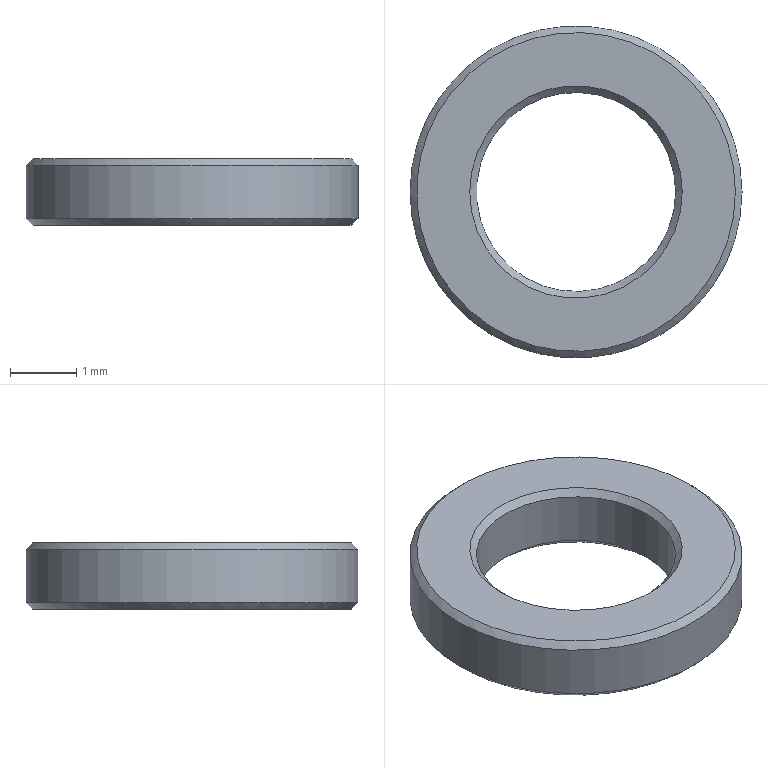Component | NX | STEPPER_WASHER | 1 solid | 15 faces | box 5 x 5 x 1 mm | volume 10 mm3 | cone 8 | cylinder 4 | plane 3 | commonest cylinder face diameters 5 x1 3 x1 4.5 x1 3.5 x1
STEP:
#1=CARTESIAN_POINT('',(0.,0.,0.));
#2=DIRECTION('',(0.,0.,1.));
#3=DIRECTION('',(1.,0.,0.));
#4=AXIS2_PLACEMENT_3D('',#1,#2,#3);
#5=CARTESIAN_POINT('',(2.4,0.,11.2));
#6=VERTEX_POINT('',#5);
#7=CARTESIAN_POINT('',(0.,0.,11.2));
#8=DIRECTION('',(0.,0.,-1.));
#9=DIRECTION('',(1.,0.,0.));
#10=AXIS2_PLACEMENT_3D('',#7,#8,#9);
#11=CIRCLE('',#10,2.4);
#12=CARTESIAN_POINT('',(0.,0.,11.2));
#13=DIRECTION('',(0.,0.,-1.));
#14=DIRECTION('',(1.,0.,0.));
#15=AXIS2_PLACEMENT_3D('',#12,#13,#14);
#16=PLANE('',#15);
#17=CARTESIAN_POINT('',(0.,0.));
#18=DIRECTION('',(1.,0.));
#19=AXIS2_PLACEMENT_2D('',#17,#18);
#20=CIRCLE('',#19,2.4);
#21=(GEOMETRIC_REPRESENTATION_CONTEXT(2)PARAMETRIC_REPRESENTATION_CONTEXT()REPRESENTATION_CONTEXT('',''));
#22=DEFINITIONAL_REPRESENTATION('',(#20),#21);
#23=PCURVE('',#16,#22);
#24=CARTESIAN_POINT('',(0.,0.,11.2));
#25=DIRECTION('',(0.,0.,1.));
#26=DIRECTION('',(-1.,0.,0.));
#27=AXIS2_PLACEMENT_3D('',#24,#25,#26);
#28=CONICAL_SURFACE('',#27,2.4,0.7854);
#29=CARTESIAN_POINT('',(9.425,0.));
#30=DIRECTION('',(-1.,0.));
#31=VECTOR('',#30,1.);
#32=LINE('',#29,#31);
#33=(GEOMETRIC_REPRESENTATION_CONTEXT(2)PARAMETRIC_REPRESENTATION_CONTEXT()REPRESENTATION_CONTEXT('',''));
#34=DEFINITIONAL_REPRESENTATION('',(#32),#33);
#35=PCURVE('',#28,#34);
#36=SURFACE_CURVE('',#11,(#23,#35),.PCURVE_S1.);
#37=EDGE_CURVE('',#6,#6,#36,.T.);
#38=ORIENTED_EDGE('',*,*,#37,.T.);
#39=EDGE_LOOP('',(#38));
#40=FACE_BOUND('',#39,.T.);
#41=CARTESIAN_POINT('',(2.35,0.,11.2));
#42=VERTEX_POINT('',#41);
#43=CARTESIAN_POINT('',(0.,0.,11.2));
#44=DIRECTION('',(0.,0.,1.));
#45=DIRECTION('',(1.,0.,0.));
#46=AXIS2_PLACEMENT_3D('',#43,#44,#45);
#47=CIRCLE('',#46,2.35);
#48=CARTESIAN_POINT('',(2.35,0.));
#49=CARTESIAN_POINT('',(2.35,-4.07));
#50=CARTESIAN_POINT('',(-1.175,-2.035));
#51=CARTESIAN_POINT('',(-4.7,-0.));
#52=CARTESIAN_POINT('',(-1.175,2.035));
#53=CARTESIAN_POINT('',(2.35,4.07));
#54=CARTESIAN_POINT('',(2.35,0.));
#55=(BOUNDED_CURVE()B_SPLINE_CURVE(2,(#48,#49,#50,#51,#52,#53,#54),.UNSPECIFIED.,.T.,.F.)B_SPLINE_CURVE_WITH_KNOTS((1,2,2,2,2,1),(-2.094,0.,2.094,4.189,6.283,8.378),.UNSPECIFIED.)CURVE()GEOMETRIC_REPRESENTATION_ITEM()RATIONAL_B_SPLINE_CURVE((1.,0.5,1.,0.5,1.,0.5,1.))REPRESENTATION_ITEM(''));
#56=(GEOMETRIC_REPRESENTATION_CONTEXT(2)PARAMETRIC_REPRESENTATION_CONTEXT()REPRESENTATION_CONTEXT('',''));
#57=DEFINITIONAL_REPRESENTATION('',(#55),#56);
#58=PCURVE('',#16,#57);
#59=CARTESIAN_POINT('',(0.,0.,11.3));
#60=DIRECTION('',(0.,0.,-1.));
#61=DIRECTION('',(1.,0.,0.));
#62=AXIS2_PLACEMENT_3D('',#59,#60,#61);
#63=CONICAL_SURFACE('',#62,2.25,0.7854);
#64=CARTESIAN_POINT('',(6.283,0.1));
#65=DIRECTION('',(-1.,0.));
#66=VECTOR('',#65,1.);
#67=LINE('',#64,#66);
#68=(GEOMETRIC_REPRESENTATION_CONTEXT(2)PARAMETRIC_REPRESENTATION_CONTEXT()REPRESENTATION_CONTEXT('',''));
#69=DEFINITIONAL_REPRESENTATION('',(#67),#68);
#70=PCURVE('',#63,#69);
#71=SURFACE_CURVE('',#47,(#58,#70),.PCURVE_S1.);
#72=EDGE_CURVE('',#42,#42,#71,.T.);
#73=ORIENTED_EDGE('',*,*,#72,.T.);
#74=EDGE_LOOP('',(#73));
#75=FACE_BOUND('',#74,.T.);
#76=ADVANCED_FACE('',(#40,#75),#16,.T.);
#77=CARTESIAN_POINT('',(2.5,0.,12.1));
#78=VERTEX_POINT('',#77);
#79=CARTESIAN_POINT('',(0.,0.,12.1));
#80=DIRECTION('',(0.,0.,-1.));
#81=DIRECTION('',(1.,0.,0.));
#82=AXIS2_PLACEMENT_3D('',#79,#80,#81);
#83=CIRCLE('',#82,2.5);
#84=CARTESIAN_POINT('',(0.,0.,11.2));
#85=DIRECTION('',(0.,0.,1.));
#86=DIRECTION('',(-1.,0.,0.));
#87=AXIS2_PLACEMENT_3D('',#84,#85,#86);
#88=CYLINDRICAL_SURFACE('',#87,2.5);
#89=CARTESIAN_POINT('',(9.425,0.9));
#90=DIRECTION('',(-1.,0.));
#91=VECTOR('',#90,1.);
#92=LINE('',#89,#91);
#93=(GEOMETRIC_REPRESENTATION_CONTEXT(2)PARAMETRIC_REPRESENTATION_CONTEXT()REPRESENTATION_CONTEXT('',''));
#94=DEFINITIONAL_REPRESENTATION('',(#92),#93);
#95=PCURVE('',#88,#94);
#96=CARTESIAN_POINT('',(0.,0.,12.1));
#97=DIRECTION('',(0.,0.,-1.));
#98=DIRECTION('',(1.,0.,0.));
#99=AXIS2_PLACEMENT_3D('',#96,#97,#98);
#100=CONICAL_SURFACE('',#99,2.5,0.7854);
#101=CARTESIAN_POINT('',(0.,0.));
#102=DIRECTION('',(1.,0.));
#103=VECTOR('',#102,1.);
#104=LINE('',#101,#103);
#105=(GEOMETRIC_REPRESENTATION_CONTEXT(2)PARAMETRIC_REPRESENTATION_CONTEXT()REPRESENTATION_CONTEXT('',''));
#106=DEFINITIONAL_REPRESENTATION('',(#104),#105);
#107=PCURVE('',#100,#106);
#108=SURFACE_CURVE('',#83,(#95,#107),.PCURVE_S1.);
#109=EDGE_CURVE('',#78,#78,#108,.T.);
#110=ORIENTED_EDGE('',*,*,#109,.T.);
#111=CARTESIAN_POINT('',(2.5,0.,11.3));
#112=VERTEX_POINT('',#111);
#113=CARTESIAN_POINT('',(2.5,-0.,11.3));
#114=CARTESIAN_POINT('',(2.5,-0.,12.1));
#115=B_SPLINE_CURVE_WITH_KNOTS('',1,(#113,#114),.UNSPECIFIED.,.F.,.F.,(2,2),(0.1,0.9),.PIECEWISE_BEZIER_KNOTS.);
#116=CARTESIAN_POINT('',(3.142,0.));
#117=DIRECTION('',(0.,1.));
#118=VECTOR('',#117,1.);
#119=LINE('',#116,#118);
#120=(GEOMETRIC_REPRESENTATION_CONTEXT(2)PARAMETRIC_REPRESENTATION_CONTEXT()REPRESENTATION_CONTEXT('',''));
#121=DEFINITIONAL_REPRESENTATION('',(#119),#120);
#122=PCURVE('',#88,#121);
#123=CARTESIAN_POINT('',(9.425,0.));
#124=DIRECTION('',(0.,1.));
#125=VECTOR('',#124,1.);
#126=LINE('',#123,#125);
#127=(GEOMETRIC_REPRESENTATION_CONTEXT(2)PARAMETRIC_REPRESENTATION_CONTEXT()REPRESENTATION_CONTEXT('',''));
#128=DEFINITIONAL_REPRESENTATION('',(#126),#127);
#129=PCURVE('',#88,#128);
#130=SEAM_CURVE('',#115,(#122,#129),.PCURVE_S1.);
#131=EDGE_CURVE('',#112,#78,#130,.T.);
#132=ORIENTED_EDGE('',*,*,#131,.F.);
#133=CARTESIAN_POINT('',(0.,0.,11.3));
#134=DIRECTION('',(0.,0.,1.));
#135=DIRECTION('',(1.,0.,0.));
#136=AXIS2_PLACEMENT_3D('',#133,#134,#135);
#137=CIRCLE('',#136,2.5);
#138=CARTESIAN_POINT('',(3.142,0.1));
#139=DIRECTION('',(1.,0.));
#140=VECTOR('',#139,1.);
#141=LINE('',#138,#140);
#142=(GEOMETRIC_REPRESENTATION_CONTEXT(2)PARAMETRIC_REPRESENTATION_CONTEXT()REPRESENTATION_CONTEXT('',''));
#143=DEFINITIONAL_REPRESENTATION('',(#141),#142);
#144=PCURVE('',#88,#143);
#145=CARTESIAN_POINT('',(3.142,0.1));
#146=DIRECTION('',(1.,0.));
#147=VECTOR('',#146,1.);
#148=LINE('',#145,#147);
#149=(GEOMETRIC_REPRESENTATION_CONTEXT(2)PARAMETRIC_REPRESENTATION_CONTEXT()REPRESENTATION_CONTEXT('',''));
#150=DEFINITIONAL_REPRESENTATION('',(#148),#149);
#151=PCURVE('',#28,#150);
#152=SURFACE_CURVE('',#137,(#144,#151),.PCURVE_S1.);
#153=EDGE_CURVE('',#112,#112,#152,.T.);
#154=ORIENTED_EDGE('',*,*,#153,.T.);
#155=ORIENTED_EDGE('',*,*,#131,.T.);
#156=EDGE_LOOP('',(#110,#132,#154,#155));
#157=FACE_BOUND('',#156,.T.);
#158=ADVANCED_FACE('',(#157),#88,.T.);
#159=CARTESIAN_POINT('',(1.5,0.,12.1));
#160=VERTEX_POINT('',#159);
#161=CARTESIAN_POINT('',(0.,0.,12.1));
#162=DIRECTION('',(0.,0.,1.));
#163=DIRECTION('',(1.,0.,0.));
#164=AXIS2_PLACEMENT_3D('',#161,#162,#163);
#165=CIRCLE('',#164,1.5);
#166=CARTESIAN_POINT('',(0.,0.,11.2));
#167=DIRECTION('',(0.,0.,1.));
#168=DIRECTION('',(-1.,0.,0.));
#169=AXIS2_PLACEMENT_3D('',#166,#167,#168);
#170=CYLINDRICAL_SURFACE('',#169,1.5);
#171=CARTESIAN_POINT('',(3.142,0.9));
#172=DIRECTION('',(1.,0.));
#173=VECTOR('',#172,1.);
#174=LINE('',#171,#173);
#175=(GEOMETRIC_REPRESENTATION_CONTEXT(2)PARAMETRIC_REPRESENTATION_CONTEXT()REPRESENTATION_CONTEXT('',''));
#176=DEFINITIONAL_REPRESENTATION('',(#174),#175);
#177=PCURVE('',#170,#176);
#178=CARTESIAN_POINT('',(0.,0.,12.2));
#179=DIRECTION('',(0.,0.,1.));
#180=DIRECTION('',(-1.,0.,0.));
#181=AXIS2_PLACEMENT_3D('',#178,#179,#180);
#182=CONICAL_SURFACE('',#181,1.6,0.7854);
#183=CARTESIAN_POINT('',(3.142,-0.1));
#184=DIRECTION('',(1.,0.));
#185=VECTOR('',#184,1.);
#186=LINE('',#183,#185);
#187=(GEOMETRIC_REPRESENTATION_CONTEXT(2)PARAMETRIC_REPRESENTATION_CONTEXT()REPRESENTATION_CONTEXT('',''));
#188=DEFINITIONAL_REPRESENTATION('',(#186),#187);
#189=PCURVE('',#182,#188);
#190=SURFACE_CURVE('',#165,(#177,#189),.PCURVE_S1.);
#191=EDGE_CURVE('',#160,#160,#190,.T.);
#192=ORIENTED_EDGE('',*,*,#191,.F.);
#193=CARTESIAN_POINT('',(1.5,0.,11.3));
#194=VERTEX_POINT('',#193);
#195=CARTESIAN_POINT('',(1.5,-0.,11.3));
#196=CARTESIAN_POINT('',(1.5,-0.,12.1));
#197=B_SPLINE_CURVE_WITH_KNOTS('',1,(#195,#196),.UNSPECIFIED.,.F.,.F.,(2,2),(0.1,0.9),.PIECEWISE_BEZIER_KNOTS.);
#198=CARTESIAN_POINT('',(3.142,0.));
#199=DIRECTION('',(0.,1.));
#200=VECTOR('',#199,1.);
#201=LINE('',#198,#200);
#202=(GEOMETRIC_REPRESENTATION_CONTEXT(2)PARAMETRIC_REPRESENTATION_CONTEXT()REPRESENTATION_CONTEXT('',''));
#203=DEFINITIONAL_REPRESENTATION('',(#201),#202);
#204=PCURVE('',#170,#203);
#205=CARTESIAN_POINT('',(9.425,0.));
#206=DIRECTION('',(0.,1.));
#207=VECTOR('',#206,1.);
#208=LINE('',#205,#207);
#209=(GEOMETRIC_REPRESENTATION_CONTEXT(2)PARAMETRIC_REPRESENTATION_CONTEXT()REPRESENTATION_CONTEXT('',''));
#210=DEFINITIONAL_REPRESENTATION('',(#208),#209);
#211=PCURVE('',#170,#210);
#212=SEAM_CURVE('',#197,(#204,#211),.PCURVE_S1.);
#213=EDGE_CURVE('',#194,#160,#212,.T.);
#214=ORIENTED_EDGE('',*,*,#213,.F.);
#215=CARTESIAN_POINT('',(0.,0.,11.3));
#216=DIRECTION('',(0.,0.,-1.));
#217=DIRECTION('',(1.,0.,0.));
#218=AXIS2_PLACEMENT_3D('',#215,#216,#217);
#219=CIRCLE('',#218,1.5);
#220=CARTESIAN_POINT('',(9.425,0.1));
#221=DIRECTION('',(-1.,0.));
#222=VECTOR('',#221,1.);
#223=LINE('',#220,#222);
#224=(GEOMETRIC_REPRESENTATION_CONTEXT(2)PARAMETRIC_REPRESENTATION_CONTEXT()REPRESENTATION_CONTEXT('',''));
#225=DEFINITIONAL_REPRESENTATION('',(#223),#224);
#226=PCURVE('',#170,#225);
#227=CARTESIAN_POINT('',(0.,0.,11.3));
#228=DIRECTION('',(0.,0.,-1.));
#229=DIRECTION('',(1.,0.,0.));
#230=AXIS2_PLACEMENT_3D('',#227,#228,#229);
#231=CONICAL_SURFACE('',#230,1.5,0.7854);
#232=CARTESIAN_POINT('',(0.,0.));
#233=DIRECTION('',(1.,0.));
#234=VECTOR('',#233,1.);
#235=LINE('',#232,#234);
#236=(GEOMETRIC_REPRESENTATION_CONTEXT(2)PARAMETRIC_REPRESENTATION_CONTEXT()REPRESENTATION_CONTEXT('',''));
#237=DEFINITIONAL_REPRESENTATION('',(#235),#236);
#238=PCURVE('',#231,#237);
#239=SURFACE_CURVE('',#219,(#226,#238),.PCURVE_S1.);
#240=EDGE_CURVE('',#194,#194,#239,.T.);
#241=ORIENTED_EDGE('',*,*,#240,.F.);
#242=ORIENTED_EDGE('',*,*,#213,.T.);
#243=EDGE_LOOP('',(#192,#214,#241,#242));
#244=FACE_BOUND('',#243,.F.);
#245=ADVANCED_FACE('',(#244),#170,.F.);
#246=CARTESIAN_POINT('',(1.6,0.,11.2));
#247=VERTEX_POINT('',#246);
#248=CARTESIAN_POINT('',(0.,0.,11.2));
#249=DIRECTION('',(0.,0.,1.));
#250=DIRECTION('',(1.,0.,0.));
#251=AXIS2_PLACEMENT_3D('',#248,#249,#250);
#252=CIRCLE('',#251,1.6);
#253=CARTESIAN_POINT('',(0.,0.,11.2));
#254=DIRECTION('',(0.,0.,-1.));
#255=DIRECTION('',(1.,0.,0.));
#256=AXIS2_PLACEMENT_3D('',#253,#254,#255);
#257=PLANE('',#256);
#258=CARTESIAN_POINT('',(1.6,0.));
#259=CARTESIAN_POINT('',(1.6,-2.771));
#260=CARTESIAN_POINT('',(-0.8,-1.386));
#261=CARTESIAN_POINT('',(-3.2,-0.));
#262=CARTESIAN_POINT('',(-0.8,1.386));
#263=CARTESIAN_POINT('',(1.6,2.771));
#264=CARTESIAN_POINT('',(1.6,0.));
#265=(BOUNDED_CURVE()B_SPLINE_CURVE(2,(#258,#259,#260,#261,#262,#263,#264),.UNSPECIFIED.,.T.,.F.)B_SPLINE_CURVE_WITH_KNOTS((1,2,2,2,2,1),(-2.094,0.,2.094,4.189,6.283,8.378),.UNSPECIFIED.)CURVE()GEOMETRIC_REPRESENTATION_ITEM()RATIONAL_B_SPLINE_CURVE((1.,0.5,1.,0.5,1.,0.5,1.))REPRESENTATION_ITEM(''));
#266=(GEOMETRIC_REPRESENTATION_CONTEXT(2)PARAMETRIC_REPRESENTATION_CONTEXT()REPRESENTATION_CONTEXT('',''));
#267=DEFINITIONAL_REPRESENTATION('',(#265),#266);
#268=PCURVE('',#257,#267);
#269=CARTESIAN_POINT('',(6.283,0.1));
#270=DIRECTION('',(-1.,0.));
#271=VECTOR('',#270,1.);
#272=LINE('',#269,#271);
#273=(GEOMETRIC_REPRESENTATION_CONTEXT(2)PARAMETRIC_REPRESENTATION_CONTEXT()REPRESENTATION_CONTEXT('',''));
#274=DEFINITIONAL_REPRESENTATION('',(#272),#273);
#275=PCURVE('',#231,#274);
#276=SURFACE_CURVE('',#252,(#268,#275),.PCURVE_S1.);
#277=EDGE_CURVE('',#247,#247,#276,.T.);
#278=ORIENTED_EDGE('',*,*,#277,.T.);
#279=EDGE_LOOP('',(#278));
#280=FACE_BOUND('',#279,.T.);
#281=CARTESIAN_POINT('',(1.65,0.,11.2));
#282=VERTEX_POINT('',#281);
#283=CARTESIAN_POINT('',(0.,0.,11.2));
#284=DIRECTION('',(0.,0.,-1.));
#285=DIRECTION('',(1.,0.,0.));
#286=AXIS2_PLACEMENT_3D('',#283,#284,#285);
#287=CIRCLE('',#286,1.65);
#288=CARTESIAN_POINT('',(0.,0.));
#289=DIRECTION('',(1.,0.));
#290=AXIS2_PLACEMENT_2D('',#288,#289);
#291=CIRCLE('',#290,1.65);
#292=(GEOMETRIC_REPRESENTATION_CONTEXT(2)PARAMETRIC_REPRESENTATION_CONTEXT()REPRESENTATION_CONTEXT('',''));
#293=DEFINITIONAL_REPRESENTATION('',(#291),#292);
#294=PCURVE('',#257,#293);
#295=CARTESIAN_POINT('',(0.,0.,11.3));
#296=DIRECTION('',(0.,0.,1.));
#297=DIRECTION('',(-1.,0.,0.));
#298=AXIS2_PLACEMENT_3D('',#295,#296,#297);
#299=CONICAL_SURFACE('',#298,1.75,0.7854);
#300=CARTESIAN_POINT('',(9.425,-0.1));
#301=DIRECTION('',(-1.,0.));
#302=VECTOR('',#301,1.);
#303=LINE('',#300,#302);
#304=(GEOMETRIC_REPRESENTATION_CONTEXT(2)PARAMETRIC_REPRESENTATION_CONTEXT()REPRESENTATION_CONTEXT('',''));
#305=DEFINITIONAL_REPRESENTATION('',(#303),#304);
#306=PCURVE('',#299,#305);
#307=SURFACE_CURVE('',#287,(#294,#306),.PCURVE_S1.);
#308=EDGE_CURVE('',#282,#282,#307,.T.);
#309=ORIENTED_EDGE('',*,*,#308,.T.);
#310=EDGE_LOOP('',(#309));
#311=FACE_BOUND('',#310,.T.);
#312=ADVANCED_FACE('',(#280,#311),#257,.T.);
#313=CARTESIAN_POINT('',(1.6,0.,12.2));
#314=VERTEX_POINT('',#313);
#315=CARTESIAN_POINT('',(0.,0.,12.2));
#316=DIRECTION('',(0.,0.,-1.));
#317=DIRECTION('',(1.,0.,0.));
#318=AXIS2_PLACEMENT_3D('',#315,#316,#317);
#319=CIRCLE('',#318,1.6);
#320=CARTESIAN_POINT('',(0.,0.,12.2));
#321=DIRECTION('',(0.,0.,-1.));
#322=DIRECTION('',(1.,0.,0.));
#323=AXIS2_PLACEMENT_3D('',#320,#321,#322);
#324=PLANE('',#323);
#325=CARTESIAN_POINT('',(0.,0.));
#326=DIRECTION('',(1.,0.));
#327=AXIS2_PLACEMENT_2D('',#325,#326);
#328=CIRCLE('',#327,1.6);
#329=(GEOMETRIC_REPRESENTATION_CONTEXT(2)PARAMETRIC_REPRESENTATION_CONTEXT()REPRESENTATION_CONTEXT('',''));
#330=DEFINITIONAL_REPRESENTATION('',(#328),#329);
#331=PCURVE('',#324,#330);
#332=CARTESIAN_POINT('',(9.425,0.));
#333=DIRECTION('',(-1.,0.));
#334=VECTOR('',#333,1.);
#335=LINE('',#332,#334);
#336=(GEOMETRIC_REPRESENTATION_CONTEXT(2)PARAMETRIC_REPRESENTATION_CONTEXT()REPRESENTATION_CONTEXT('',''));
#337=DEFINITIONAL_REPRESENTATION('',(#335),#336);
#338=PCURVE('',#182,#337);
#339=SURFACE_CURVE('',#319,(#331,#338),.PCURVE_S1.);
#340=EDGE_CURVE('',#314,#314,#339,.T.);
#341=ORIENTED_EDGE('',*,*,#340,.T.);
#342=EDGE_LOOP('',(#341));
#343=FACE_BOUND('',#342,.T.);
#344=CARTESIAN_POINT('',(2.4,0.,12.2));
#345=VERTEX_POINT('',#344);
#346=CARTESIAN_POINT('',(0.,0.,12.2));
#347=DIRECTION('',(0.,0.,1.));
#348=DIRECTION('',(1.,0.,0.));
#349=AXIS2_PLACEMENT_3D('',#346,#347,#348);
#350=CIRCLE('',#349,2.4);
#351=CARTESIAN_POINT('',(2.4,0.));
#352=CARTESIAN_POINT('',(2.4,-4.157));
#353=CARTESIAN_POINT('',(-1.2,-2.078));
#354=CARTESIAN_POINT('',(-4.8,-0.));
#355=CARTESIAN_POINT('',(-1.2,2.078));
#356=CARTESIAN_POINT('',(2.4,4.157));
#357=CARTESIAN_POINT('',(2.4,0.));
#358=(BOUNDED_CURVE()B_SPLINE_CURVE(2,(#351,#352,#353,#354,#355,#356,#357),.UNSPECIFIED.,.T.,.F.)B_SPLINE_CURVE_WITH_KNOTS((1,2,2,2,2,1),(-2.094,0.,2.094,4.189,6.283,8.378),.UNSPECIFIED.)CURVE()GEOMETRIC_REPRESENTATION_ITEM()RATIONAL_B_SPLINE_CURVE((1.,0.5,1.,0.5,1.,0.5,1.))REPRESENTATION_ITEM(''));
#359=(GEOMETRIC_REPRESENTATION_CONTEXT(2)PARAMETRIC_REPRESENTATION_CONTEXT()REPRESENTATION_CONTEXT('',''));
#360=DEFINITIONAL_REPRESENTATION('',(#358),#359);
#361=PCURVE('',#324,#360);
#362=CARTESIAN_POINT('',(6.283,-0.1));
#363=DIRECTION('',(-1.,0.));
#364=VECTOR('',#363,1.);
#365=LINE('',#362,#364);
#366=(GEOMETRIC_REPRESENTATION_CONTEXT(2)PARAMETRIC_REPRESENTATION_CONTEXT()REPRESENTATION_CONTEXT('',''));
#367=DEFINITIONAL_REPRESENTATION('',(#365),#366);
#368=PCURVE('',#100,#367);
#369=SURFACE_CURVE('',#350,(#361,#368),.PCURVE_S1.);
#370=EDGE_CURVE('',#345,#345,#369,.T.);
#371=ORIENTED_EDGE('',*,*,#370,.T.);
#372=EDGE_LOOP('',(#371));
#373=FACE_BOUND('',#372,.T.);
#374=ADVANCED_FACE('',(#343,#373),#324,.F.);
#375=CARTESIAN_POINT('',(2.25,0.,11.3));
#376=VERTEX_POINT('',#375);
#377=CARTESIAN_POINT('',(0.,0.,11.3));
#378=DIRECTION('',(0.,0.,-1.));
#379=DIRECTION('',(1.,0.,0.));
#380=AXIS2_PLACEMENT_3D('',#377,#378,#379);
#381=CIRCLE('',#380,2.25);
#382=CARTESIAN_POINT('',(0.,0.,11.7));
#383=DIRECTION('',(0.,0.,-1.));
#384=DIRECTION('',(1.,0.,0.));
#385=AXIS2_PLACEMENT_3D('',#382,#383,#384);
#386=CYLINDRICAL_SURFACE('',#385,2.25);
#387=CARTESIAN_POINT('',(0.,0.4));
#388=DIRECTION('',(1.,0.));
#389=VECTOR('',#388,1.);
#390=LINE('',#387,#389);
#391=(GEOMETRIC_REPRESENTATION_CONTEXT(2)PARAMETRIC_REPRESENTATION_CONTEXT()REPRESENTATION_CONTEXT('',''));
#392=DEFINITIONAL_REPRESENTATION('',(#390),#391);
#393=PCURVE('',#386,#392);
#394=CARTESIAN_POINT('',(0.,0.));
#395=DIRECTION('',(1.,0.));
#396=VECTOR('',#395,1.);
#397=LINE('',#394,#396);
#398=(GEOMETRIC_REPRESENTATION_CONTEXT(2)PARAMETRIC_REPRESENTATION_CONTEXT()REPRESENTATION_CONTEXT('',''));
#399=DEFINITIONAL_REPRESENTATION('',(#397),#398);
#400=PCURVE('',#63,#399);
#401=SURFACE_CURVE('',#381,(#393,#400),.PCURVE_S1.);
#402=EDGE_CURVE('',#376,#376,#401,.T.);
#403=ORIENTED_EDGE('',*,*,#402,.F.);
#404=CARTESIAN_POINT('',(2.25,0.,11.45));
#405=VERTEX_POINT('',#404);
#406=CARTESIAN_POINT('',(2.25,0.,11.45));
#407=CARTESIAN_POINT('',(2.25,0.,11.3));
#408=B_SPLINE_CURVE_WITH_KNOTS('',1,(#406,#407),.UNSPECIFIED.,.F.,.F.,(2,2),(0.25,0.4),.PIECEWISE_BEZIER_KNOTS.);
#409=CARTESIAN_POINT('',(0.,0.));
#410=DIRECTION('',(0.,1.));
#411=VECTOR('',#410,1.);
#412=LINE('',#409,#411);
#413=(GEOMETRIC_REPRESENTATION_CONTEXT(2)PARAMETRIC_REPRESENTATION_CONTEXT()REPRESENTATION_CONTEXT('',''));
#414=DEFINITIONAL_REPRESENTATION('',(#412),#413);
#415=PCURVE('',#386,#414);
#416=CARTESIAN_POINT('',(6.283,0.));
#417=DIRECTION('',(0.,1.));
#418=VECTOR('',#417,1.);
#419=LINE('',#416,#418);
#420=(GEOMETRIC_REPRESENTATION_CONTEXT(2)PARAMETRIC_REPRESENTATION_CONTEXT()REPRESENTATION_CONTEXT('',''));
#421=DEFINITIONAL_REPRESENTATION('',(#419),#420);
#422=PCURVE('',#386,#421);
#423=SEAM_CURVE('',#408,(#415,#422),.PCURVE_S1.);
#424=EDGE_CURVE('',#405,#376,#423,.T.);
#425=ORIENTED_EDGE('',*,*,#424,.F.);
#426=CARTESIAN_POINT('',(0.,0.,11.45));
#427=DIRECTION('',(0.,0.,1.));
#428=DIRECTION('',(1.,0.,0.));
#429=AXIS2_PLACEMENT_3D('',#426,#427,#428);
#430=CIRCLE('',#429,2.25);
#431=CARTESIAN_POINT('',(6.283,0.25));
#432=DIRECTION('',(-1.,0.));
#433=VECTOR('',#432,1.);
#434=LINE('',#431,#433);
#435=(GEOMETRIC_REPRESENTATION_CONTEXT(2)PARAMETRIC_REPRESENTATION_CONTEXT()REPRESENTATION_CONTEXT('',''));
#436=DEFINITIONAL_REPRESENTATION('',(#434),#435);
#437=PCURVE('',#386,#436);
#438=CARTESIAN_POINT('',(0.,0.,11.45));
#439=DIRECTION('',(0.,0.,-1.));
#440=DIRECTION('',(1.,0.,0.));
#441=AXIS2_PLACEMENT_3D('',#438,#439,#440);
#442=CONICAL_SURFACE('',#441,2.25,0.7854);
#443=CARTESIAN_POINT('',(6.283,0.));
#444=DIRECTION('',(-1.,0.));
#445=VECTOR('',#444,1.);
#446=LINE('',#443,#445);
#447=(GEOMETRIC_REPRESENTATION_CONTEXT(2)PARAMETRIC_REPRESENTATION_CONTEXT()REPRESENTATION_CONTEXT('',''));
#448=DEFINITIONAL_REPRESENTATION('',(#446),#447);
#449=PCURVE('',#442,#448);
#450=SURFACE_CURVE('',#430,(#437,#449),.PCURVE_S1.);
#451=EDGE_CURVE('',#405,#405,#450,.T.);
#452=ORIENTED_EDGE('',*,*,#451,.F.);
#453=ORIENTED_EDGE('',*,*,#424,.T.);
#454=EDGE_LOOP('',(#403,#425,#452,#453));
#455=FACE_BOUND('',#454,.F.);
#456=ADVANCED_FACE('',(#455),#386,.F.);
#457=CARTESIAN_POINT('',(1.75,0.,11.3));
#458=VERTEX_POINT('',#457);
#459=CARTESIAN_POINT('',(0.,0.,11.3));
#460=DIRECTION('',(0.,0.,1.));
#461=DIRECTION('',(1.,0.,0.));
#462=AXIS2_PLACEMENT_3D('',#459,#460,#461);
#463=CIRCLE('',#462,1.75);
#464=CARTESIAN_POINT('',(0.,0.,11.7));
#465=DIRECTION('',(0.,0.,-1.));
#466=DIRECTION('',(1.,0.,0.));
#467=AXIS2_PLACEMENT_3D('',#464,#465,#466);
#468=CYLINDRICAL_SURFACE('',#467,1.75);
#469=CARTESIAN_POINT('',(6.283,0.4));
#470=DIRECTION('',(-1.,0.));
#471=VECTOR('',#470,1.);
#472=LINE('',#469,#471);
#473=(GEOMETRIC_REPRESENTATION_CONTEXT(2)PARAMETRIC_REPRESENTATION_CONTEXT()REPRESENTATION_CONTEXT('',''));
#474=DEFINITIONAL_REPRESENTATION('',(#472),#473);
#475=PCURVE('',#468,#474);
#476=CARTESIAN_POINT('',(3.142,0.));
#477=DIRECTION('',(1.,0.));
#478=VECTOR('',#477,1.);
#479=LINE('',#476,#478);
#480=(GEOMETRIC_REPRESENTATION_CONTEXT(2)PARAMETRIC_REPRESENTATION_CONTEXT()REPRESENTATION_CONTEXT('',''));
#481=DEFINITIONAL_REPRESENTATION('',(#479),#480);
#482=PCURVE('',#299,#481);
#483=SURFACE_CURVE('',#463,(#475,#482),.PCURVE_S1.);
#484=EDGE_CURVE('',#458,#458,#483,.T.);
#485=ORIENTED_EDGE('',*,*,#484,.T.);
#486=CARTESIAN_POINT('',(1.75,0.,11.45));
#487=VERTEX_POINT('',#486);
#488=CARTESIAN_POINT('',(1.75,0.,11.45));
#489=CARTESIAN_POINT('',(1.75,0.,11.3));
#490=B_SPLINE_CURVE_WITH_KNOTS('',1,(#488,#489),.UNSPECIFIED.,.F.,.F.,(2,2),(0.25,0.4),.PIECEWISE_BEZIER_KNOTS.);
#491=CARTESIAN_POINT('',(0.,0.));
#492=DIRECTION('',(0.,1.));
#493=VECTOR('',#492,1.);
#494=LINE('',#491,#493);
#495=(GEOMETRIC_REPRESENTATION_CONTEXT(2)PARAMETRIC_REPRESENTATION_CONTEXT()REPRESENTATION_CONTEXT('',''));
#496=DEFINITIONAL_REPRESENTATION('',(#494),#495);
#497=PCURVE('',#468,#496);
#498=CARTESIAN_POINT('',(6.283,0.));
#499=DIRECTION('',(0.,1.));
#500=VECTOR('',#499,1.);
#501=LINE('',#498,#500);
#502=(GEOMETRIC_REPRESENTATION_CONTEXT(2)PARAMETRIC_REPRESENTATION_CONTEXT()REPRESENTATION_CONTEXT('',''));
#503=DEFINITIONAL_REPRESENTATION('',(#501),#502);
#504=PCURVE('',#468,#503);
#505=SEAM_CURVE('',#490,(#497,#504),.PCURVE_S1.);
#506=EDGE_CURVE('',#487,#458,#505,.T.);
#507=ORIENTED_EDGE('',*,*,#506,.F.);
#508=CARTESIAN_POINT('',(0.,0.,11.45));
#509=DIRECTION('',(0.,0.,-1.));
#510=DIRECTION('',(1.,0.,0.));
#511=AXIS2_PLACEMENT_3D('',#508,#509,#510);
#512=CIRCLE('',#511,1.75);
#513=CARTESIAN_POINT('',(0.,0.25));
#514=DIRECTION('',(1.,0.));
#515=VECTOR('',#514,1.);
#516=LINE('',#513,#515);
#517=(GEOMETRIC_REPRESENTATION_CONTEXT(2)PARAMETRIC_REPRESENTATION_CONTEXT()REPRESENTATION_CONTEXT('',''));
#518=DEFINITIONAL_REPRESENTATION('',(#516),#517);
#519=PCURVE('',#468,#518);
#520=CARTESIAN_POINT('',(0.,0.,11.45));
#521=DIRECTION('',(0.,0.,1.));
#522=DIRECTION('',(-1.,0.,0.));
#523=AXIS2_PLACEMENT_3D('',#520,#521,#522);
#524=CONICAL_SURFACE('',#523,1.75,0.7854);
#525=CARTESIAN_POINT('',(9.425,0.));
#526=DIRECTION('',(-1.,0.));
#527=VECTOR('',#526,1.);
#528=LINE('',#525,#527);
#529=(GEOMETRIC_REPRESENTATION_CONTEXT(2)PARAMETRIC_REPRESENTATION_CONTEXT()REPRESENTATION_CONTEXT('',''));
#530=DEFINITIONAL_REPRESENTATION('',(#528),#529);
#531=PCURVE('',#524,#530);
#532=SURFACE_CURVE('',#512,(#519,#531),.PCURVE_S1.);
#533=EDGE_CURVE('',#487,#487,#532,.T.);
#534=ORIENTED_EDGE('',*,*,#533,.T.);
#535=ORIENTED_EDGE('',*,*,#506,.T.);
#536=EDGE_LOOP('',(#485,#507,#534,#535));
#537=FACE_BOUND('',#536,.T.);
#538=ADVANCED_FACE('',(#537),#468,.T.);
#539=ORIENTED_EDGE('',*,*,#451,.T.);
#540=CARTESIAN_POINT('',(2.,0.,11.7));
#541=VERTEX_POINT('',#540);
#542=CARTESIAN_POINT('',(2.,0.,11.7));
#543=CARTESIAN_POINT('',(2.25,0.,11.45));
#544=B_SPLINE_CURVE_WITH_KNOTS('',1,(#542,#543),.UNSPECIFIED.,.F.,.F.,(2,2),(-0.3536,0.),.PIECEWISE_BEZIER_KNOTS.);
#545=CARTESIAN_POINT('',(0.,0.));
#546=DIRECTION('',(0.,1.));
#547=VECTOR('',#546,1.);
#548=LINE('',#545,#547);
#549=(GEOMETRIC_REPRESENTATION_CONTEXT(2)PARAMETRIC_REPRESENTATION_CONTEXT()REPRESENTATION_CONTEXT('',''));
#550=DEFINITIONAL_REPRESENTATION('',(#548),#549);
#551=PCURVE('',#442,#550);
#552=CARTESIAN_POINT('',(6.283,0.));
#553=DIRECTION('',(0.,1.));
#554=VECTOR('',#553,1.);
#555=LINE('',#552,#554);
#556=(GEOMETRIC_REPRESENTATION_CONTEXT(2)PARAMETRIC_REPRESENTATION_CONTEXT()REPRESENTATION_CONTEXT('',''));
#557=DEFINITIONAL_REPRESENTATION('',(#555),#556);
#558=PCURVE('',#442,#557);
#559=SEAM_CURVE('',#544,(#551,#558),.PCURVE_S1.);
#560=EDGE_CURVE('',#541,#405,#559,.T.);
#561=ORIENTED_EDGE('',*,*,#560,.F.);
#562=CARTESIAN_POINT('',(0.,0.,11.7));
#563=DIRECTION('',(0.,0.,-1.));
#564=DIRECTION('',(1.,0.,0.));
#565=AXIS2_PLACEMENT_3D('',#562,#563,#564);
#566=CIRCLE('',#565,2.);
#567=CARTESIAN_POINT('',(0.,-0.25));
#568=DIRECTION('',(1.,0.));
#569=VECTOR('',#568,1.);
#570=LINE('',#567,#569);
#571=(GEOMETRIC_REPRESENTATION_CONTEXT(2)PARAMETRIC_REPRESENTATION_CONTEXT()REPRESENTATION_CONTEXT('',''));
#572=DEFINITIONAL_REPRESENTATION('',(#570),#571);
#573=PCURVE('',#442,#572);
#574=CARTESIAN_POINT('',(9.425,0.25));
#575=DIRECTION('',(-1.,0.));
#576=VECTOR('',#575,1.);
#577=LINE('',#574,#576);
#578=(GEOMETRIC_REPRESENTATION_CONTEXT(2)PARAMETRIC_REPRESENTATION_CONTEXT()REPRESENTATION_CONTEXT('',''));
#579=DEFINITIONAL_REPRESENTATION('',(#577),#578);
#580=PCURVE('',#524,#579);
#581=SURFACE_CURVE('',#566,(#573,#580),.PCURVE_S1.);
#582=EDGE_CURVE('',#541,#541,#581,.T.);
#583=ORIENTED_EDGE('',*,*,#582,.T.);
#584=ORIENTED_EDGE('',*,*,#560,.T.);
#585=EDGE_LOOP('',(#539,#561,#583,#584));
#586=FACE_BOUND('',#585,.F.);
#587=ADVANCED_FACE('',(#586),#442,.F.);
#588=ORIENTED_EDGE('',*,*,#582,.T.);
#589=CARTESIAN_POINT('',(1.75,-0.,11.45));
#590=CARTESIAN_POINT('',(2.,-0.,11.7));
#591=B_SPLINE_CURVE_WITH_KNOTS('',1,(#589,#590),.UNSPECIFIED.,.F.,.F.,(2,2),(0.,0.3536),.PIECEWISE_BEZIER_KNOTS.);
#592=CARTESIAN_POINT('',(3.142,0.));
#593=DIRECTION('',(0.,1.));
#594=VECTOR('',#593,1.);
#595=LINE('',#592,#594);
#596=(GEOMETRIC_REPRESENTATION_CONTEXT(2)PARAMETRIC_REPRESENTATION_CONTEXT()REPRESENTATION_CONTEXT('',''));
#597=DEFINITIONAL_REPRESENTATION('',(#595),#596);
#598=PCURVE('',#524,#597);
#599=CARTESIAN_POINT('',(9.425,0.));
#600=DIRECTION('',(0.,1.));
#601=VECTOR('',#600,1.);
#602=LINE('',#599,#601);
#603=(GEOMETRIC_REPRESENTATION_CONTEXT(2)PARAMETRIC_REPRESENTATION_CONTEXT()REPRESENTATION_CONTEXT('',''));
#604=DEFINITIONAL_REPRESENTATION('',(#602),#603);
#605=PCURVE('',#524,#604);
#606=SEAM_CURVE('',#591,(#598,#605),.PCURVE_S1.);
#607=EDGE_CURVE('',#487,#541,#606,.T.);
#608=ORIENTED_EDGE('',*,*,#607,.F.);
#609=ORIENTED_EDGE('',*,*,#533,.F.);
#610=ORIENTED_EDGE('',*,*,#607,.T.);
#611=EDGE_LOOP('',(#588,#608,#609,#610));
#612=FACE_BOUND('',#611,.T.);
#613=ADVANCED_FACE('',(#612),#524,.T.);
#614=ORIENTED_EDGE('',*,*,#191,.T.);
#615=CARTESIAN_POINT('',(1.5,-0.,12.1));
#616=CARTESIAN_POINT('',(1.6,-0.,12.2));
#617=B_SPLINE_CURVE_WITH_KNOTS('',1,(#615,#616),.UNSPECIFIED.,.F.,.F.,(2,2),(-0.1414,0.),.PIECEWISE_BEZIER_KNOTS.);
#618=CARTESIAN_POINT('',(9.425,0.));
#619=DIRECTION('',(0.,1.));
#620=VECTOR('',#619,1.);
#621=LINE('',#618,#620);
#622=(GEOMETRIC_REPRESENTATION_CONTEXT(2)PARAMETRIC_REPRESENTATION_CONTEXT()REPRESENTATION_CONTEXT('',''));
#623=DEFINITIONAL_REPRESENTATION('',(#621),#622);
#624=PCURVE('',#182,#623);
#625=CARTESIAN_POINT('',(3.142,0.));
#626=DIRECTION('',(0.,1.));
#627=VECTOR('',#626,1.);
#628=LINE('',#625,#627);
#629=(GEOMETRIC_REPRESENTATION_CONTEXT(2)PARAMETRIC_REPRESENTATION_CONTEXT()REPRESENTATION_CONTEXT('',''));
#630=DEFINITIONAL_REPRESENTATION('',(#628),#629);
#631=PCURVE('',#182,#630);
#632=SEAM_CURVE('',#617,(#624,#631),.PCURVE_S1.);
#633=EDGE_CURVE('',#160,#314,#632,.T.);
#634=ORIENTED_EDGE('',*,*,#633,.T.);
#635=ORIENTED_EDGE('',*,*,#340,.T.);
#636=ORIENTED_EDGE('',*,*,#633,.F.);
#637=EDGE_LOOP('',(#614,#634,#635,#636));
#638=FACE_BOUND('',#637,.F.);
#639=ADVANCED_FACE('',(#638),#182,.F.);
#640=ORIENTED_EDGE('',*,*,#370,.F.);
#641=CARTESIAN_POINT('',(2.4,0.,12.2));
#642=CARTESIAN_POINT('',(2.5,0.,12.1));
#643=B_SPLINE_CURVE_WITH_KNOTS('',1,(#641,#642),.UNSPECIFIED.,.F.,.F.,(2,2),(-0.1414,0.),.PIECEWISE_BEZIER_KNOTS.);
#644=CARTESIAN_POINT('',(6.283,0.));
#645=DIRECTION('',(0.,1.));
#646=VECTOR('',#645,1.);
#647=LINE('',#644,#646);
#648=(GEOMETRIC_REPRESENTATION_CONTEXT(2)PARAMETRIC_REPRESENTATION_CONTEXT()REPRESENTATION_CONTEXT('',''));
#649=DEFINITIONAL_REPRESENTATION('',(#647),#648);
#650=PCURVE('',#100,#649);
#651=CARTESIAN_POINT('',(0.,0.));
#652=DIRECTION('',(0.,1.));
#653=VECTOR('',#652,1.);
#654=LINE('',#651,#653);
#655=(GEOMETRIC_REPRESENTATION_CONTEXT(2)PARAMETRIC_REPRESENTATION_CONTEXT()REPRESENTATION_CONTEXT('',''));
#656=DEFINITIONAL_REPRESENTATION('',(#654),#655);
#657=PCURVE('',#100,#656);
#658=SEAM_CURVE('',#643,(#650,#657),.PCURVE_S1.);
#659=EDGE_CURVE('',#345,#78,#658,.T.);
#660=ORIENTED_EDGE('',*,*,#659,.T.);
#661=ORIENTED_EDGE('',*,*,#109,.F.);
#662=ORIENTED_EDGE('',*,*,#659,.F.);
#663=EDGE_LOOP('',(#640,#660,#661,#662));
#664=FACE_BOUND('',#663,.T.);
#665=ADVANCED_FACE('',(#664),#100,.T.);
#666=ORIENTED_EDGE('',*,*,#277,.T.);
#667=CARTESIAN_POINT('',(1.5,0.,11.3));
#668=CARTESIAN_POINT('',(1.6,0.,11.2));
#669=B_SPLINE_CURVE_WITH_KNOTS('',1,(#667,#668),.UNSPECIFIED.,.F.,.F.,(2,2),(0.,0.1414),.PIECEWISE_BEZIER_KNOTS.);
#670=CARTESIAN_POINT('',(0.,0.));
#671=DIRECTION('',(0.,1.));
#672=VECTOR('',#671,1.);
#673=LINE('',#670,#672);
#674=(GEOMETRIC_REPRESENTATION_CONTEXT(2)PARAMETRIC_REPRESENTATION_CONTEXT()REPRESENTATION_CONTEXT('',''));
#675=DEFINITIONAL_REPRESENTATION('',(#673),#674);
#676=PCURVE('',#231,#675);
#677=CARTESIAN_POINT('',(6.283,0.));
#678=DIRECTION('',(0.,1.));
#679=VECTOR('',#678,1.);
#680=LINE('',#677,#679);
#681=(GEOMETRIC_REPRESENTATION_CONTEXT(2)PARAMETRIC_REPRESENTATION_CONTEXT()REPRESENTATION_CONTEXT('',''));
#682=DEFINITIONAL_REPRESENTATION('',(#680),#681);
#683=PCURVE('',#231,#682);
#684=SEAM_CURVE('',#669,(#676,#683),.PCURVE_S1.);
#685=EDGE_CURVE('',#194,#247,#684,.T.);
#686=ORIENTED_EDGE('',*,*,#685,.F.);
#687=ORIENTED_EDGE('',*,*,#240,.T.);
#688=ORIENTED_EDGE('',*,*,#685,.T.);
#689=EDGE_LOOP('',(#666,#686,#687,#688));
#690=FACE_BOUND('',#689,.F.);
#691=ADVANCED_FACE('',(#690),#231,.F.);
#692=ORIENTED_EDGE('',*,*,#308,.F.);
#693=CARTESIAN_POINT('',(1.65,-0.,11.2));
#694=CARTESIAN_POINT('',(1.75,-0.,11.3));
#695=B_SPLINE_CURVE_WITH_KNOTS('',1,(#693,#694),.UNSPECIFIED.,.F.,.F.,(2,2),(-0.1414,0.),.PIECEWISE_BEZIER_KNOTS.);
#696=CARTESIAN_POINT('',(9.425,0.));
#697=DIRECTION('',(0.,1.));
#698=VECTOR('',#697,1.);
#699=LINE('',#696,#698);
#700=(GEOMETRIC_REPRESENTATION_CONTEXT(2)PARAMETRIC_REPRESENTATION_CONTEXT()REPRESENTATION_CONTEXT('',''));
#701=DEFINITIONAL_REPRESENTATION('',(#699),#700);
#702=PCURVE('',#299,#701);
#703=CARTESIAN_POINT('',(3.142,0.));
#704=DIRECTION('',(0.,1.));
#705=VECTOR('',#704,1.);
#706=LINE('',#703,#705);
#707=(GEOMETRIC_REPRESENTATION_CONTEXT(2)PARAMETRIC_REPRESENTATION_CONTEXT()REPRESENTATION_CONTEXT('',''));
#708=DEFINITIONAL_REPRESENTATION('',(#706),#707);
#709=PCURVE('',#299,#708);
#710=SEAM_CURVE('',#695,(#702,#709),.PCURVE_S1.);
#711=EDGE_CURVE('',#282,#458,#710,.T.);
#712=ORIENTED_EDGE('',*,*,#711,.T.);
#713=ORIENTED_EDGE('',*,*,#484,.F.);
#714=ORIENTED_EDGE('',*,*,#711,.F.);
#715=EDGE_LOOP('',(#692,#712,#713,#714));
#716=FACE_BOUND('',#715,.T.);
#717=ADVANCED_FACE('',(#716),#299,.T.);
#718=ORIENTED_EDGE('',*,*,#153,.F.);
#719=CARTESIAN_POINT('',(2.4,-0.,11.2));
#720=CARTESIAN_POINT('',(2.5,-0.,11.3));
#721=B_SPLINE_CURVE_WITH_KNOTS('',1,(#719,#720),.UNSPECIFIED.,.F.,.F.,(2,2),(0.,0.1414),.PIECEWISE_BEZIER_KNOTS.);
#722=CARTESIAN_POINT('',(3.142,0.));
#723=DIRECTION('',(0.,1.));
#724=VECTOR('',#723,1.);
#725=LINE('',#722,#724);
#726=(GEOMETRIC_REPRESENTATION_CONTEXT(2)PARAMETRIC_REPRESENTATION_CONTEXT()REPRESENTATION_CONTEXT('',''));
#727=DEFINITIONAL_REPRESENTATION('',(#725),#726);
#728=PCURVE('',#28,#727);
#729=CARTESIAN_POINT('',(9.425,0.));
#730=DIRECTION('',(0.,1.));
#731=VECTOR('',#730,1.);
#732=LINE('',#729,#731);
#733=(GEOMETRIC_REPRESENTATION_CONTEXT(2)PARAMETRIC_REPRESENTATION_CONTEXT()REPRESENTATION_CONTEXT('',''));
#734=DEFINITIONAL_REPRESENTATION('',(#732),#733);
#735=PCURVE('',#28,#734);
#736=SEAM_CURVE('',#721,(#728,#735),.PCURVE_S1.);
#737=EDGE_CURVE('',#6,#112,#736,.T.);
#738=ORIENTED_EDGE('',*,*,#737,.F.);
#739=ORIENTED_EDGE('',*,*,#37,.F.);
#740=ORIENTED_EDGE('',*,*,#737,.T.);
#741=EDGE_LOOP('',(#718,#738,#739,#740));
#742=FACE_BOUND('',#741,.T.);
#743=ADVANCED_FACE('',(#742),#28,.T.);
#744=ORIENTED_EDGE('',*,*,#72,.T.);
#745=CARTESIAN_POINT('',(2.25,0.,11.3));
#746=CARTESIAN_POINT('',(2.35,0.,11.2));
#747=B_SPLINE_CURVE_WITH_KNOTS('',1,(#745,#746),.UNSPECIFIED.,.F.,.F.,(2,2),(0.,0.1414),.PIECEWISE_BEZIER_KNOTS.);
#748=CARTESIAN_POINT('',(0.,0.));
#749=DIRECTION('',(0.,1.));
#750=VECTOR('',#749,1.);
#751=LINE('',#748,#750);
#752=(GEOMETRIC_REPRESENTATION_CONTEXT(2)PARAMETRIC_REPRESENTATION_CONTEXT()REPRESENTATION_CONTEXT('',''));
#753=DEFINITIONAL_REPRESENTATION('',(#751),#752);
#754=PCURVE('',#63,#753);
#755=CARTESIAN_POINT('',(6.283,0.));
#756=DIRECTION('',(0.,1.));
#757=VECTOR('',#756,1.);
#758=LINE('',#755,#757);
#759=(GEOMETRIC_REPRESENTATION_CONTEXT(2)PARAMETRIC_REPRESENTATION_CONTEXT()REPRESENTATION_CONTEXT('',''));
#760=DEFINITIONAL_REPRESENTATION('',(#758),#759);
#761=PCURVE('',#63,#760);
#762=SEAM_CURVE('',#747,(#754,#761),.PCURVE_S1.);
#763=EDGE_CURVE('',#376,#42,#762,.T.);
#764=ORIENTED_EDGE('',*,*,#763,.F.);
#765=ORIENTED_EDGE('',*,*,#402,.T.);
#766=ORIENTED_EDGE('',*,*,#763,.T.);
#767=EDGE_LOOP('',(#744,#764,#765,#766));
#768=FACE_BOUND('',#767,.F.);
#769=ADVANCED_FACE('',(#768),#63,.F.);
#770=CLOSED_SHELL('',(#76,#158,#245,#312,#374,#456,#538,#587,#613,#639,#665,#691,#717,#743,#769));
#771=MANIFOLD_SOLID_BREP('',#770);
#772=(LENGTH_UNIT()NAMED_UNIT(*)SI_UNIT(.MILLI.,.METRE.));
#773=UNCERTAINTY_MEASURE_WITH_UNIT(LENGTH_MEASURE(0.00001),#772,'','');
#774=(NAMED_UNIT(*)PLANE_ANGLE_UNIT()SI_UNIT($,.RADIAN.));
#775=(NAMED_UNIT(*)SI_UNIT($,.STERADIAN.)SOLID_ANGLE_UNIT());
#776=(GEOMETRIC_REPRESENTATION_CONTEXT(3)GLOBAL_UNCERTAINTY_ASSIGNED_CONTEXT((#773))GLOBAL_UNIT_ASSIGNED_CONTEXT((#772,#774,#775))REPRESENTATION_CONTEXT('',''));
#777=ADVANCED_BREP_SHAPE_REPRESENTATION('',(#4,#771),#776);